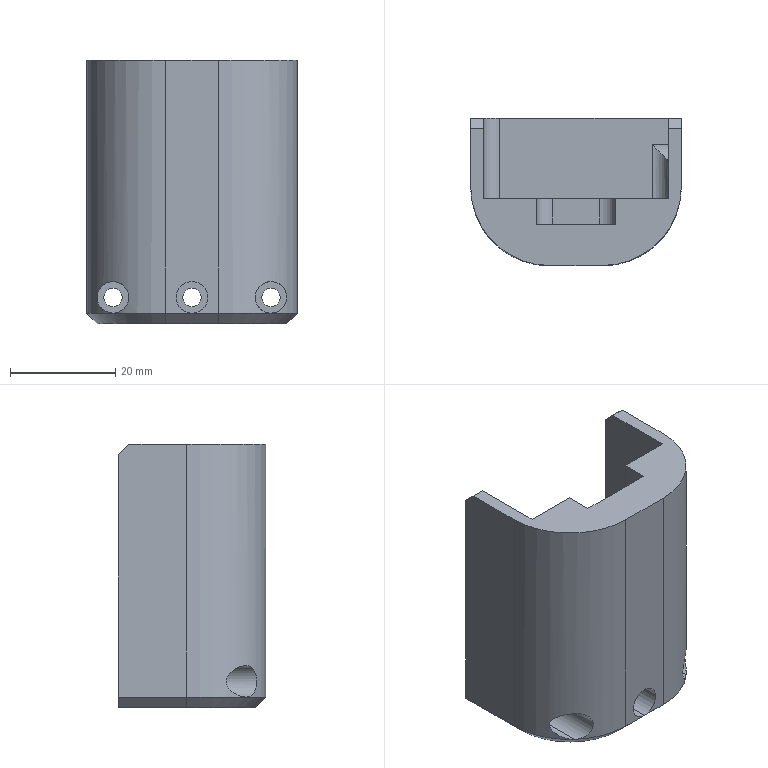Component | SolidWorks | DZ.KX.203-TC1505-20-18-05-97-1 | 1 solid | 54 faces | volume 26429 mm3 | cylinder 24 | plane 24 | cone 6 | commonest cylinder face diameters 6 x12 3.5 x6 1.6 x4 30 x2 | material Plain Carbon Steel